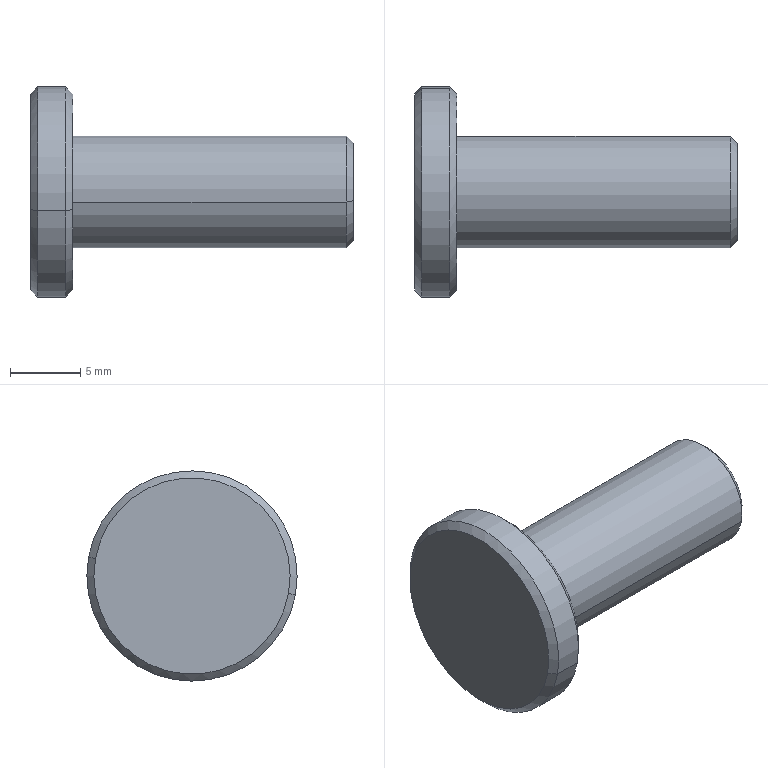Component | SolidWorks | 09HHHHHH5-1 | 1 solid | 17 faces | box 23 x 15 x 15 mm | volume 1268 mm3 | cone 8 | cylinder 6 | plane 3 | commonest cylinder face diameters 5 x2 15 x2 8 x2
build123d program:
from build123d import *

# Parameters (mm, degrees)
SKETCH1_R             = 4
BOSS_EXTRUDE1_DEPTH   = 20
SKETCH2_R             = 7.5
BOSS_EXTRUDE2_DEPTH   = 3
M5_TAPPED_HOLE1_D     = 5
M5_TAPPED_HOLE1_DEPTH = 12.4
M5_TAPPED_HOLE1_TIP   = 1.502
CHAMFER1_SIZE         = 0.5
CHAMFER2_SIZE         = 0.5


with BuildPart() as part:
    # Sketch1 → Boss-Extrude1 (new body)
    with BuildSketch(Plane.XY):
        with Locations((302.287, -36.6)):
            Circle(SKETCH1_R)
    extrude(amount=BOSS_EXTRUDE1_DEPTH)

    # Sketch2 → Boss-Extrude2 (add)
    with BuildSketch(Plane.XY.offset(20)):
        with Locations((302.287, -36.6)):
            Circle(SKETCH2_R)
    extrude(amount=BOSS_EXTRUDE2_DEPTH)

    # M5 Tapped Hole1
    with Locations(Plane(origin=(0, 0, 0), x_dir=(-1, 0, 0), z_dir=(0, 0, -1))):
        with Locations((-302.287, -36.6)):
            Hole(M5_TAPPED_HOLE1_D / 2, depth=M5_TAPPED_HOLE1_DEPTH)
            with Locations((0, 0, -(M5_TAPPED_HOLE1_DEPTH + M5_TAPPED_HOLE1_TIP / 2))):  # 118° drill point
                Cone(0, M5_TAPPED_HOLE1_D / 2, M5_TAPPED_HOLE1_TIP, mode=Mode.SUBTRACT)

    # Chamfer1
    chamfer1_edges = [part.edges().sort_by_distance(p)[0] for p in [
        (294.787, -36.6, 20),
        (294.787, -36.6, 23),
    ]]
    chamfer(chamfer1_edges, length=CHAMFER1_SIZE)

    # Chamfer2
    chamfer2_edges = [part.edges().sort_by_distance(p)[0] for p in [
        (298.287, -36.6, 0),
    ]]
    chamfer(chamfer2_edges, length=CHAMFER2_SIZE)


solid = part.part

# Placed as in the assembly
solid = solid.moved(Location((-649.859, -249.783, -332.543), (0, -90, 0)))
STEP:
#1=COLOUR_RGB('',0.7922,0.8196,0.9333);
#2=FILL_AREA_STYLE_COLOUR('',#1);
#3=FILL_AREA_STYLE('',(#2));
#4=SURFACE_STYLE_FILL_AREA(#3);
#5=SURFACE_SIDE_STYLE('',(#4));
#6=SURFACE_STYLE_USAGE(.BOTH.,#5);
#7=PRESENTATION_STYLE_ASSIGNMENT((#6));
#8=CARTESIAN_POINT('',(-25.585,-11.139,-1.167));
#9=VERTEX_POINT('',#8);
#10=CARTESIAN_POINT('',(-25.585,-11.411,-1.216));
#11=VERTEX_POINT('',#10);
#12=CARTESIAN_POINT('',(-25.585,-11.275,-1.191));
#13=DIRECTION('',(1.,-0.,0.));
#14=DIRECTION('',(0.,-0.9839,-0.1787));
#15=AXIS2_PLACEMENT_3D('',#12,#13,#14);
#16=CIRCLE('',#15,0.1378);
#17=EDGE_CURVE('',#9,#11,#16,.T.);
#18=ORIENTED_EDGE('',*,*,#17,.F.);
#19=CARTESIAN_POINT('',(-25.605,-11.12,-1.163));
#20=VERTEX_POINT('',#19);
#21=CARTESIAN_POINT('',(-25.605,-11.12,-1.163));
#22=DIRECTION('',(-0.7071,0.6957,0.1264));
#23=VECTOR('',#22,39.37);
#24=LINE('',#21,#23);
#25=EDGE_CURVE('',#9,#20,#24,.T.);
#26=ORIENTED_EDGE('',*,*,#25,.T.);
#27=CARTESIAN_POINT('',(-25.605,-11.43,-1.219));
#28=VERTEX_POINT('',#27);
#29=CARTESIAN_POINT('',(-25.605,-11.275,-1.191));
#30=DIRECTION('',(-1.,0.,-0.));
#31=DIRECTION('',(0.,-0.9839,-0.1787));
#32=AXIS2_PLACEMENT_3D('',#29,#30,#31);
#33=CIRCLE('',#32,0.1575);
#34=EDGE_CURVE('',#28,#20,#33,.T.);
#35=ORIENTED_EDGE('',*,*,#34,.F.);
#36=CARTESIAN_POINT('',(-25.605,-11.43,-1.219));
#37=DIRECTION('',(-0.7071,-0.6957,-0.1264));
#38=VECTOR('',#37,39.37);
#39=LINE('',#36,#38);
#40=EDGE_CURVE('',#11,#28,#39,.T.);
#41=ORIENTED_EDGE('',*,*,#40,.F.);
#42=EDGE_LOOP('',(#18,#26,#35,#41));
#43=FACE_OUTER_BOUND('',#42,.T.);
#44=CARTESIAN_POINT('',(-25.605,-11.275,-1.191));
#45=DIRECTION('',(-1.,0.,-0.));
#46=DIRECTION('',(0.,-0.9839,-0.1787));
#47=AXIS2_PLACEMENT_3D('',#44,#45,#46);
#48=CONICAL_SURFACE('',#47,0.1575,0.7854);
#49=ADVANCED_FACE('',(#43),#48,.T.);
#50=CARTESIAN_POINT('',(-26.372,-11.004,-1.142));
#51=VERTEX_POINT('',#50);
#52=CARTESIAN_POINT('',(-26.372,-11.546,-1.24));
#53=VERTEX_POINT('',#52);
#54=CARTESIAN_POINT('',(-26.372,-11.275,-1.191));
#55=DIRECTION('',(1.,-0.,0.));
#56=DIRECTION('',(0.,-0.9839,-0.1787));
#57=AXIS2_PLACEMENT_3D('',#54,#55,#56);
#58=CIRCLE('',#57,0.2756);
#59=EDGE_CURVE('',#51,#53,#58,.T.);
#60=ORIENTED_EDGE('',*,*,#59,.F.);
#61=CARTESIAN_POINT('',(-26.392,-10.984,-1.138));
#62=VERTEX_POINT('',#61);
#63=CARTESIAN_POINT('',(-26.392,-10.984,-1.138));
#64=DIRECTION('',(-0.7071,0.6957,0.1264));
#65=VECTOR('',#64,39.37);
#66=LINE('',#63,#65);
#67=EDGE_CURVE('',#51,#62,#66,.T.);
#68=ORIENTED_EDGE('',*,*,#67,.T.);
#69=CARTESIAN_POINT('',(-26.392,-11.565,-1.244));
#70=VERTEX_POINT('',#69);
#71=CARTESIAN_POINT('',(-26.392,-11.275,-1.191));
#72=DIRECTION('',(-1.,0.,-0.));
#73=DIRECTION('',(0.,-0.9839,-0.1787));
#74=AXIS2_PLACEMENT_3D('',#71,#72,#73);
#75=CIRCLE('',#74,0.2953);
#76=EDGE_CURVE('',#70,#62,#75,.T.);
#77=ORIENTED_EDGE('',*,*,#76,.F.);
#78=CARTESIAN_POINT('',(-26.392,-11.565,-1.244));
#79=DIRECTION('',(-0.7071,-0.6957,-0.1264));
#80=VECTOR('',#79,39.37);
#81=LINE('',#78,#80);
#82=EDGE_CURVE('',#53,#70,#81,.T.);
#83=ORIENTED_EDGE('',*,*,#82,.F.);
#84=EDGE_LOOP('',(#60,#68,#77,#83));
#85=FACE_OUTER_BOUND('',#84,.T.);
#86=CARTESIAN_POINT('',(-26.392,-11.275,-1.191));
#87=DIRECTION('',(-1.,0.,-0.));
#88=DIRECTION('',(0.,-0.9839,-0.1787));
#89=AXIS2_PLACEMENT_3D('',#86,#87,#88);
#90=CONICAL_SURFACE('',#89,0.2953,0.7854);
#91=ADVANCED_FACE('',(#85),#90,.T.);
#92=CARTESIAN_POINT('',(-26.491,-11.546,-1.24));
#93=VERTEX_POINT('',#92);
#94=CARTESIAN_POINT('',(-26.491,-11.004,-1.142));
#95=VERTEX_POINT('',#94);
#96=CARTESIAN_POINT('',(-26.491,-11.275,-1.191));
#97=DIRECTION('',(-1.,0.,-0.));
#98=DIRECTION('',(0.,-0.9839,-0.1787));
#99=AXIS2_PLACEMENT_3D('',#96,#97,#98);
#100=CIRCLE('',#99,0.2756);
#101=EDGE_CURVE('',#93,#95,#100,.T.);
#102=ORIENTED_EDGE('',*,*,#101,.F.);
#103=CARTESIAN_POINT('',(-26.471,-11.565,-1.244));
#104=VERTEX_POINT('',#103);
#105=CARTESIAN_POINT('',(-26.491,-11.546,-1.24));
#106=DIRECTION('',(0.7071,-0.6957,-0.1264));
#107=VECTOR('',#106,39.37);
#108=LINE('',#105,#107);
#109=EDGE_CURVE('',#93,#104,#108,.T.);
#110=ORIENTED_EDGE('',*,*,#109,.T.);
#111=CARTESIAN_POINT('',(-26.471,-10.984,-1.138));
#112=VERTEX_POINT('',#111);
#113=CARTESIAN_POINT('',(-26.471,-11.275,-1.191));
#114=DIRECTION('',(1.,-0.,0.));
#115=DIRECTION('',(0.,-0.9839,-0.1787));
#116=AXIS2_PLACEMENT_3D('',#113,#114,#115);
#117=CIRCLE('',#116,0.2953);
#118=EDGE_CURVE('',#112,#104,#117,.T.);
#119=ORIENTED_EDGE('',*,*,#118,.F.);
#120=CARTESIAN_POINT('',(-26.491,-11.004,-1.142));
#121=DIRECTION('',(0.7071,0.6957,0.1264));
#122=VECTOR('',#121,39.37);
#123=LINE('',#120,#122);
#124=EDGE_CURVE('',#95,#112,#123,.T.);
#125=ORIENTED_EDGE('',*,*,#124,.F.);
#126=EDGE_LOOP('',(#102,#110,#119,#125));
#127=FACE_OUTER_BOUND('',#126,.T.);
#128=CARTESIAN_POINT('',(-26.491,-11.275,-1.191));
#129=DIRECTION('',(1.,-0.,0.));
#130=DIRECTION('',(0.,0.9839,0.1787));
#131=AXIS2_PLACEMENT_3D('',#128,#129,#130);
#132=CONICAL_SURFACE('',#131,0.2756,0.7854);
#133=ADVANCED_FACE('',(#127),#132,.T.);
#134=CARTESIAN_POINT('',(-26.073,-11.372,-1.209));
#135=VERTEX_POINT('',#134);
#136=CARTESIAN_POINT('',(-26.073,-11.178,-1.174));
#137=VERTEX_POINT('',#136);
#138=CARTESIAN_POINT('',(-26.073,-11.275,-1.191));
#139=DIRECTION('',(1.,-0.,0.));
#140=DIRECTION('',(0.,0.9839,0.1787));
#141=AXIS2_PLACEMENT_3D('',#138,#139,#140);
#142=CIRCLE('',#141,0.09843);
#143=EDGE_CURVE('',#135,#137,#142,.T.);
#144=ORIENTED_EDGE('',*,*,#143,.F.);
#145=CARTESIAN_POINT('',(-25.585,-11.372,-1.209));
#146=VERTEX_POINT('',#145);
#147=CARTESIAN_POINT('',(-25.585,-11.372,-1.209));
#148=DIRECTION('',(1.,-0.,0.));
#149=VECTOR('',#148,39.37);
#150=LINE('',#147,#149);
#151=EDGE_CURVE('',#135,#146,#150,.T.);
#152=ORIENTED_EDGE('',*,*,#151,.T.);
#153=CARTESIAN_POINT('',(-25.585,-11.178,-1.174));
#154=VERTEX_POINT('',#153);
#155=CARTESIAN_POINT('',(-25.585,-11.275,-1.191));
#156=DIRECTION('',(1.,-0.,0.));
#157=DIRECTION('',(0.,0.9839,0.1787));
#158=AXIS2_PLACEMENT_3D('',#155,#156,#157);
#159=CIRCLE('',#158,0.09843);
#160=EDGE_CURVE('',#146,#154,#159,.T.);
#161=ORIENTED_EDGE('',*,*,#160,.T.);
#162=CARTESIAN_POINT('',(-25.585,-11.178,-1.174));
#163=DIRECTION('',(1.,-0.,0.));
#164=VECTOR('',#163,39.37);
#165=LINE('',#162,#164);
#166=EDGE_CURVE('',#137,#154,#165,.T.);
#167=ORIENTED_EDGE('',*,*,#166,.F.);
#168=EDGE_LOOP('',(#144,#152,#161,#167));
#169=FACE_OUTER_BOUND('',#168,.T.);
#170=CARTESIAN_POINT('',(-25.585,-11.275,-1.191));
#171=DIRECTION('',(1.,-0.,0.));
#172=DIRECTION('',(0.,0.9839,0.1787));
#173=AXIS2_PLACEMENT_3D('',#170,#171,#172);
#174=CYLINDRICAL_SURFACE('',#173,0.09843);
#175=ADVANCED_FACE('',(#169),#174,.F.);
#176=CARTESIAN_POINT('',(-26.132,-11.275,-1.191));
#177=VERTEX_POINT('',#176);
#178=CARTESIAN_POINT('',(-26.073,-11.178,-1.174));
#179=DIRECTION('',(0.515,0.8434,0.1532));
#180=VECTOR('',#179,39.37);
#181=LINE('',#178,#180);
#182=EDGE_CURVE('',#177,#137,#181,.T.);
#183=ORIENTED_EDGE('',*,*,#182,.F.);
#184=CARTESIAN_POINT('',(-26.073,-11.372,-1.209));
#185=DIRECTION('',(0.515,-0.8434,-0.1532));
#186=VECTOR('',#185,39.37);
#187=LINE('',#184,#186);
#188=EDGE_CURVE('',#177,#135,#187,.T.);
#189=ORIENTED_EDGE('',*,*,#188,.T.);
#190=ORIENTED_EDGE('',*,*,#143,.T.);
#191=EDGE_LOOP('',(#183,#189,#190));
#192=FACE_OUTER_BOUND('',#191,.T.);
#193=CARTESIAN_POINT('',(-26.073,-11.275,-1.191));
#194=DIRECTION('',(1.,-0.,0.));
#195=DIRECTION('',(0.,0.9839,0.1787));
#196=AXIS2_PLACEMENT_3D('',#193,#194,#195);
#197=CONICAL_SURFACE('',#196,0.09843,1.03);
#198=ADVANCED_FACE('',(#192),#197,.F.);
#199=ORIENTED_EDGE('',*,*,#118,.T.);
#200=CARTESIAN_POINT('',(-26.491,-11.565,-1.244));
#201=DIRECTION('',(1.,-0.,0.));
#202=VECTOR('',#201,39.37);
#203=LINE('',#200,#202);
#204=EDGE_CURVE('',#104,#70,#203,.T.);
#205=ORIENTED_EDGE('',*,*,#204,.T.);
#206=ORIENTED_EDGE('',*,*,#76,.T.);
#207=CARTESIAN_POINT('',(-26.491,-10.984,-1.138));
#208=DIRECTION('',(1.,-0.,0.));
#209=VECTOR('',#208,39.37);
#210=LINE('',#207,#209);
#211=EDGE_CURVE('',#112,#62,#210,.T.);
#212=ORIENTED_EDGE('',*,*,#211,.F.);
#213=EDGE_LOOP('',(#199,#205,#206,#212));
#214=FACE_OUTER_BOUND('',#213,.T.);
#215=CARTESIAN_POINT('',(-26.491,-11.275,-1.191));
#216=DIRECTION('',(1.,-0.,0.));
#217=DIRECTION('',(0.,0.9839,0.1787));
#218=AXIS2_PLACEMENT_3D('',#215,#216,#217);
#219=CYLINDRICAL_SURFACE('',#218,0.2953);
#220=ADVANCED_FACE('',(#214),#219,.T.);
#221=CARTESIAN_POINT('',(-26.372,-11.43,-1.219));
#222=VERTEX_POINT('',#221);
#223=CARTESIAN_POINT('',(-26.372,-11.12,-1.163));
#224=VERTEX_POINT('',#223);
#225=CARTESIAN_POINT('',(-26.372,-11.275,-1.191));
#226=DIRECTION('',(-1.,0.,-0.));
#227=DIRECTION('',(0.,-0.9839,-0.1787));
#228=AXIS2_PLACEMENT_3D('',#225,#226,#227);
#229=CIRCLE('',#228,0.1575);
#230=EDGE_CURVE('',#222,#224,#229,.T.);
#231=ORIENTED_EDGE('',*,*,#230,.F.);
#232=CARTESIAN_POINT('',(-26.372,-11.43,-1.219));
#233=DIRECTION('',(1.,-0.,0.));
#234=VECTOR('',#233,39.37);
#235=LINE('',#232,#234);
#236=EDGE_CURVE('',#222,#28,#235,.T.);
#237=ORIENTED_EDGE('',*,*,#236,.T.);
#238=ORIENTED_EDGE('',*,*,#34,.T.);
#239=CARTESIAN_POINT('',(-26.372,-11.12,-1.163));
#240=DIRECTION('',(1.,-0.,0.));
#241=VECTOR('',#240,39.37);
#242=LINE('',#239,#241);
#243=EDGE_CURVE('',#224,#20,#242,.T.);
#244=ORIENTED_EDGE('',*,*,#243,.F.);
#245=EDGE_LOOP('',(#231,#237,#238,#244));
#246=FACE_OUTER_BOUND('',#245,.T.);
#247=CARTESIAN_POINT('',(-26.372,-11.275,-1.191));
#248=DIRECTION('',(1.,-0.,0.));
#249=DIRECTION('',(0.,0.9839,0.1787));
#250=AXIS2_PLACEMENT_3D('',#247,#248,#249);
#251=CYLINDRICAL_SURFACE('',#250,0.1575);
#252=ADVANCED_FACE('',(#246),#251,.T.);
#253=ORIENTED_EDGE('',*,*,#236,.F.);
#254=CARTESIAN_POINT('',(-26.372,-11.275,-1.191));
#255=DIRECTION('',(-1.,0.,-0.));
#256=DIRECTION('',(0.,-0.9839,-0.1787));
#257=AXIS2_PLACEMENT_3D('',#254,#255,#256);
#258=CIRCLE('',#257,0.1575);
#259=EDGE_CURVE('',#224,#222,#258,.T.);
#260=ORIENTED_EDGE('',*,*,#259,.F.);
#261=ORIENTED_EDGE('',*,*,#243,.T.);
#262=CARTESIAN_POINT('',(-25.605,-11.275,-1.191));
#263=DIRECTION('',(-1.,0.,-0.));
#264=DIRECTION('',(0.,-0.9839,-0.1787));
#265=AXIS2_PLACEMENT_3D('',#262,#263,#264);
#266=CIRCLE('',#265,0.1575);
#267=EDGE_CURVE('',#20,#28,#266,.T.);
#268=ORIENTED_EDGE('',*,*,#267,.T.);
#269=EDGE_LOOP('',(#253,#260,#261,#268));
#270=FACE_OUTER_BOUND('',#269,.T.);
#271=CARTESIAN_POINT('',(-26.372,-11.275,-1.191));
#272=DIRECTION('',(1.,-0.,0.));
#273=DIRECTION('',(0.,0.9839,0.1787));
#274=AXIS2_PLACEMENT_3D('',#271,#272,#273);
#275=CYLINDRICAL_SURFACE('',#274,0.1575);
#276=ADVANCED_FACE('',(#270),#275,.T.);
#277=CARTESIAN_POINT('',(-25.585,-11.275,-1.191));
#278=DIRECTION('',(1.,-0.,0.));
#279=DIRECTION('',(0.,-0.9839,-0.1787));
#280=AXIS2_PLACEMENT_3D('',#277,#278,#279);
#281=CIRCLE('',#280,0.1378);
#282=EDGE_CURVE('',#11,#9,#281,.T.);
#283=ORIENTED_EDGE('',*,*,#282,.T.);
#284=ORIENTED_EDGE('',*,*,#17,.T.);
#285=EDGE_LOOP('',(#283,#284));
#286=FACE_OUTER_BOUND('',#285,.T.);
#287=CARTESIAN_POINT('',(-25.585,-11.275,-1.191));
#288=DIRECTION('',(1.,-0.,0.));
#289=DIRECTION('',(0.,0.9839,0.1787));
#290=AXIS2_PLACEMENT_3D('',#287,#288,#289);
#291=CIRCLE('',#290,0.09843);
#292=EDGE_CURVE('',#154,#146,#291,.T.);
#293=ORIENTED_EDGE('',*,*,#292,.F.);
#294=ORIENTED_EDGE('',*,*,#160,.F.);
#295=EDGE_LOOP('',(#293,#294));
#296=FACE_BOUND('',#295,.T.);
#297=CARTESIAN_POINT('',(-25.585,-11.275,-1.191));
#298=DIRECTION('',(-1.,0.,-0.));
#299=DIRECTION('',(0.,-0.9839,-0.1787));
#300=AXIS2_PLACEMENT_3D('',#297,#298,#299);
#301=PLANE('',#300);
#302=ADVANCED_FACE('',(#286,#296),#301,.F.);
#303=CARTESIAN_POINT('',(-26.372,-11.275,-1.191));
#304=DIRECTION('',(1.,-0.,0.));
#305=DIRECTION('',(0.,-0.9839,-0.1787));
#306=AXIS2_PLACEMENT_3D('',#303,#304,#305);
#307=CIRCLE('',#306,0.2756);
#308=EDGE_CURVE('',#53,#51,#307,.T.);
#309=ORIENTED_EDGE('',*,*,#308,.T.);
#310=ORIENTED_EDGE('',*,*,#59,.T.);
#311=EDGE_LOOP('',(#309,#310));
#312=FACE_OUTER_BOUND('',#311,.T.);
#313=ORIENTED_EDGE('',*,*,#259,.T.);
#314=ORIENTED_EDGE('',*,*,#230,.T.);
#315=EDGE_LOOP('',(#313,#314));
#316=FACE_BOUND('',#315,.T.);
#317=CARTESIAN_POINT('',(-26.372,-11.275,-1.191));
#318=DIRECTION('',(-1.,0.,-0.));
#319=DIRECTION('',(0.,-0.9839,-0.1787));
#320=AXIS2_PLACEMENT_3D('',#317,#318,#319);
#321=PLANE('',#320);
#322=ADVANCED_FACE('',(#312,#316),#321,.F.);
#323=ORIENTED_EDGE('',*,*,#204,.F.);
#324=CARTESIAN_POINT('',(-26.471,-11.275,-1.191));
#325=DIRECTION('',(1.,-0.,0.));
#326=DIRECTION('',(0.,-0.9839,-0.1787));
#327=AXIS2_PLACEMENT_3D('',#324,#325,#326);
#328=CIRCLE('',#327,0.2953);
#329=EDGE_CURVE('',#104,#112,#328,.T.);
#330=ORIENTED_EDGE('',*,*,#329,.T.);
#331=ORIENTED_EDGE('',*,*,#211,.T.);
#332=CARTESIAN_POINT('',(-26.392,-11.275,-1.191));
#333=DIRECTION('',(-1.,0.,-0.));
#334=DIRECTION('',(0.,-0.9839,-0.1787));
#335=AXIS2_PLACEMENT_3D('',#332,#333,#334);
#336=CIRCLE('',#335,0.2953);
#337=EDGE_CURVE('',#62,#70,#336,.T.);
#338=ORIENTED_EDGE('',*,*,#337,.T.);
#339=EDGE_LOOP('',(#323,#330,#331,#338));
#340=FACE_OUTER_BOUND('',#339,.T.);
#341=CARTESIAN_POINT('',(-26.491,-11.275,-1.191));
#342=DIRECTION('',(1.,-0.,0.));
#343=DIRECTION('',(0.,0.9839,0.1787));
#344=AXIS2_PLACEMENT_3D('',#341,#342,#343);
#345=CYLINDRICAL_SURFACE('',#344,0.2953);
#346=ADVANCED_FACE('',(#340),#345,.T.);
#347=CARTESIAN_POINT('',(-26.491,-11.275,-1.191));
#348=DIRECTION('',(-1.,0.,-0.));
#349=DIRECTION('',(0.,-0.9839,-0.1787));
#350=AXIS2_PLACEMENT_3D('',#347,#348,#349);
#351=CIRCLE('',#350,0.2756);
#352=EDGE_CURVE('',#95,#93,#351,.T.);
#353=ORIENTED_EDGE('',*,*,#352,.T.);
#354=ORIENTED_EDGE('',*,*,#101,.T.);
#355=EDGE_LOOP('',(#353,#354));
#356=FACE_OUTER_BOUND('',#355,.T.);
#357=CARTESIAN_POINT('',(-26.491,-11.275,-1.191));
#358=DIRECTION('',(-1.,0.,-0.));
#359=DIRECTION('',(0.,-0.9839,-0.1787));
#360=AXIS2_PLACEMENT_3D('',#357,#358,#359);
#361=PLANE('',#360);
#362=ADVANCED_FACE('',(#356),#361,.T.);
#363=ORIENTED_EDGE('',*,*,#188,.F.);
#364=ORIENTED_EDGE('',*,*,#182,.T.);
#365=CARTESIAN_POINT('',(-26.073,-11.275,-1.191));
#366=DIRECTION('',(1.,-0.,0.));
#367=DIRECTION('',(0.,0.9839,0.1787));
#368=AXIS2_PLACEMENT_3D('',#365,#366,#367);
#369=CIRCLE('',#368,0.09843);
#370=EDGE_CURVE('',#137,#135,#369,.T.);
#371=ORIENTED_EDGE('',*,*,#370,.T.);
#372=EDGE_LOOP('',(#363,#364,#371));
#373=FACE_OUTER_BOUND('',#372,.T.);
#374=CARTESIAN_POINT('',(-26.073,-11.275,-1.191));
#375=DIRECTION('',(1.,-0.,0.));
#376=DIRECTION('',(0.,0.9839,0.1787));
#377=AXIS2_PLACEMENT_3D('',#374,#375,#376);
#378=CONICAL_SURFACE('',#377,0.09843,1.03);
#379=ADVANCED_FACE('',(#373),#378,.F.);
#380=ORIENTED_EDGE('',*,*,#151,.F.);
#381=ORIENTED_EDGE('',*,*,#370,.F.);
#382=ORIENTED_EDGE('',*,*,#166,.T.);
#383=ORIENTED_EDGE('',*,*,#292,.T.);
#384=EDGE_LOOP('',(#380,#381,#382,#383));
#385=FACE_OUTER_BOUND('',#384,.T.);
#386=CARTESIAN_POINT('',(-25.585,-11.275,-1.191));
#387=DIRECTION('',(1.,-0.,0.));
#388=DIRECTION('',(0.,0.9839,0.1787));
#389=AXIS2_PLACEMENT_3D('',#386,#387,#388);
#390=CYLINDRICAL_SURFACE('',#389,0.09843);
#391=ADVANCED_FACE('',(#385),#390,.F.);
#392=ORIENTED_EDGE('',*,*,#109,.F.);
#393=ORIENTED_EDGE('',*,*,#352,.F.);
#394=ORIENTED_EDGE('',*,*,#124,.T.);
#395=ORIENTED_EDGE('',*,*,#329,.F.);
#396=EDGE_LOOP('',(#392,#393,#394,#395));
#397=FACE_OUTER_BOUND('',#396,.T.);
#398=CARTESIAN_POINT('',(-26.491,-11.275,-1.191));
#399=DIRECTION('',(1.,-0.,0.));
#400=DIRECTION('',(0.,0.9839,0.1787));
#401=AXIS2_PLACEMENT_3D('',#398,#399,#400);
#402=CONICAL_SURFACE('',#401,0.2756,0.7854);
#403=ADVANCED_FACE('',(#397),#402,.T.);
#404=ORIENTED_EDGE('',*,*,#67,.F.);
#405=ORIENTED_EDGE('',*,*,#308,.F.);
#406=ORIENTED_EDGE('',*,*,#82,.T.);
#407=ORIENTED_EDGE('',*,*,#337,.F.);
#408=EDGE_LOOP('',(#404,#405,#406,#407));
#409=FACE_OUTER_BOUND('',#408,.T.);
#410=CARTESIAN_POINT('',(-26.392,-11.275,-1.191));
#411=DIRECTION('',(-1.,0.,-0.));
#412=DIRECTION('',(0.,-0.9839,-0.1787));
#413=AXIS2_PLACEMENT_3D('',#410,#411,#412);
#414=CONICAL_SURFACE('',#413,0.2953,0.7854);
#415=ADVANCED_FACE('',(#409),#414,.T.);
#416=ORIENTED_EDGE('',*,*,#25,.F.);
#417=ORIENTED_EDGE('',*,*,#282,.F.);
#418=ORIENTED_EDGE('',*,*,#40,.T.);
#419=ORIENTED_EDGE('',*,*,#267,.F.);
#420=EDGE_LOOP('',(#416,#417,#418,#419));
#421=FACE_OUTER_BOUND('',#420,.T.);
#422=CARTESIAN_POINT('',(-25.605,-11.275,-1.191));
#423=DIRECTION('',(-1.,0.,-0.));
#424=DIRECTION('',(0.,-0.9839,-0.1787));
#425=AXIS2_PLACEMENT_3D('',#422,#423,#424);
#426=CONICAL_SURFACE('',#425,0.1575,0.7854);
#427=ADVANCED_FACE('',(#421),#426,.T.);
#428=CLOSED_SHELL('',(#49,#91,#133,#175,#198,#220,#252,#276,#302,#322,#346,#362,#379,#391,#403,#415,#427));
#429=MANIFOLD_SOLID_BREP('',#428);
#430=STYLED_ITEM('',(#7),#429);
#431=PRESENTATION_LAYER_ASSIGNMENT('','',(#430));
#432=(LENGTH_UNIT()NAMED_UNIT(*)SI_UNIT($,.METRE.));
#433=LENGTH_MEASURE_WITH_UNIT(LENGTH_MEASURE(0.0254),#432);
#434=DIMENSIONAL_EXPONENTS(1.,0.,0.,0.,0.,0.,0.);
#435=(CONVERSION_BASED_UNIT('',#433)LENGTH_UNIT()NAMED_UNIT(#434));
#436=UNCERTAINTY_MEASURE_WITH_UNIT(LENGTH_MEASURE(0.00001),#435,'','');
#437=(NAMED_UNIT(*)PLANE_ANGLE_UNIT()SI_UNIT($,.RADIAN.));
#438=(NAMED_UNIT(*)SI_UNIT($,.STERADIAN.)SOLID_ANGLE_UNIT());
#439=(GEOMETRIC_REPRESENTATION_CONTEXT(3)GLOBAL_UNCERTAINTY_ASSIGNED_CONTEXT((#436))GLOBAL_UNIT_ASSIGNED_CONTEXT((#435,#437,#438))REPRESENTATION_CONTEXT('',''));
#440=MECHANICAL_DESIGN_GEOMETRIC_PRESENTATION_REPRESENTATION('',(#430),#439);
#441=CARTESIAN_POINT('',(0.,0.,0.));
#442=DIRECTION('',(0.,0.,1.));
#443=DIRECTION('',(1.,0.,0.));
#444=AXIS2_PLACEMENT_3D('',#441,#442,#443);
#445=(LENGTH_UNIT()NAMED_UNIT(*)SI_UNIT($,.METRE.));
#446=LENGTH_MEASURE_WITH_UNIT(LENGTH_MEASURE(0.0254),#445);
#447=DIMENSIONAL_EXPONENTS(1.,0.,0.,0.,0.,0.,0.);
#448=(CONVERSION_BASED_UNIT('',#446)LENGTH_UNIT()NAMED_UNIT(#447));
#449=UNCERTAINTY_MEASURE_WITH_UNIT(LENGTH_MEASURE(0.00001),#448,'','');
#450=(NAMED_UNIT(*)PLANE_ANGLE_UNIT()SI_UNIT($,.RADIAN.));
#451=(NAMED_UNIT(*)SI_UNIT($,.STERADIAN.)SOLID_ANGLE_UNIT());
#452=(GEOMETRIC_REPRESENTATION_CONTEXT(3)GLOBAL_UNCERTAINTY_ASSIGNED_CONTEXT((#449))GLOBAL_UNIT_ASSIGNED_CONTEXT((#448,#450,#451))REPRESENTATION_CONTEXT('',''));
#453=ADVANCED_BREP_SHAPE_REPRESENTATION('',(#429,#444),#452);